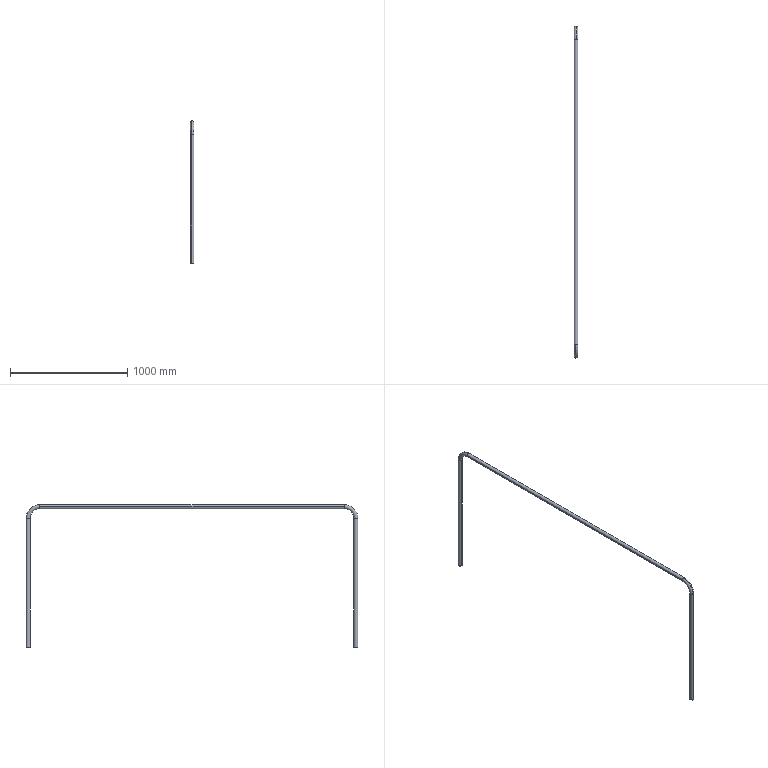Component | SolidWorks | PlatformGuardrail4-1 | 1 solid | 22 faces | box 33.5 x 2833.5 x 1216.75 mm | volume 1470094 mm3 | cylinder 12 | torus 8 | plane 2 | commonest cylinder face diameters 27.5 x6 33.5 x6 | material Plain Carbon Steel
build123d program:
from build123d import *

# Parameters (mm, degrees)
SWEEP_THIN1_PROFILE_R   = 16.75
SWEEP_THIN1_PROFILE_R_2 = 13.75


with BuildPart() as part:
    # Sweep-Thin1: sweep along a path in Sketch1
    with BuildLine(Plane(origin=(0, 0, 0), x_dir=(0, 0, -1), z_dir=(1, 0, 0))) as sweep_thin1_path:
        Line((0, 0), (0, 1100))
        ThreePointArc((0, 1100), (29.289, 1170.711), (100, 1200))
        Line((100, 1200), (2700, 1200))
        ThreePointArc((2700, 1200), (2770.711, 1170.711), (2800, 1100))
        Line((2800, 1100), (2800, 0))
    # Sweep-Thin1 profile (on start of the path) → Sweep-Thin1 (sweep)
    with BuildSketch(Plane.ZX):
        Circle(SWEEP_THIN1_PROFILE_R)
        Circle(SWEEP_THIN1_PROFILE_R_2, mode=Mode.SUBTRACT)
    sweep(path=sweep_thin1_path.line)


solid = part.part

# Placed as in the assembly
solid = solid.moved(Location((6271.051, -551.927, 5590.973), (90, 0, 0)))
STEP:
#1=COLOUR_RGB('',0.7922,0.8196,0.9333);
#2=FILL_AREA_STYLE_COLOUR('',#1);
#3=FILL_AREA_STYLE('',(#2));
#4=SURFACE_STYLE_FILL_AREA(#3);
#5=SURFACE_SIDE_STYLE('',(#4));
#6=SURFACE_STYLE_USAGE(.BOTH.,#5);
#7=PRESENTATION_STYLE_ASSIGNMENT((#6));
#8=CARTESIAN_POINT('',(247.433,84.57,267.361));
#9=VERTEX_POINT('',#8);
#10=CARTESIAN_POINT('',(246.892,84.57,267.902));
#11=VERTEX_POINT('',#10);
#12=CARTESIAN_POINT('',(246.892,84.57,267.361));
#13=DIRECTION('',(-0.,-1.,-0.));
#14=DIRECTION('',(-1.,0.,0.));
#15=AXIS2_PLACEMENT_3D('',#12,#13,#14);
#16=CIRCLE('',#15,0.5413);
#17=EDGE_CURVE('',#9,#11,#16,.T.);
#18=ORIENTED_EDGE('',*,*,#17,.T.);
#19=CARTESIAN_POINT('',(246.892,89.048,263.424));
#20=VERTEX_POINT('',#19);
#21=CARTESIAN_POINT('',(246.892,84.57,263.424));
#22=DIRECTION('',(-1.,0.,-0.));
#23=DIRECTION('',(-0.,-1.,0.));
#24=AXIS2_PLACEMENT_3D('',#21,#22,#23);
#25=CIRCLE('',#24,4.478);
#26=EDGE_CURVE('',#11,#20,#25,.T.);
#27=ORIENTED_EDGE('',*,*,#26,.T.);
#28=CARTESIAN_POINT('',(246.892,87.965,263.424));
#29=VERTEX_POINT('',#28);
#30=CARTESIAN_POINT('',(246.892,88.507,263.424));
#31=DIRECTION('',(-0.,-0.,1.));
#32=DIRECTION('',(-0.,-1.,0.));
#33=AXIS2_PLACEMENT_3D('',#30,#31,#32);
#34=CIRCLE('',#33,0.5413);
#35=EDGE_CURVE('',#29,#20,#34,.T.);
#36=ORIENTED_EDGE('',*,*,#35,.F.);
#37=CARTESIAN_POINT('',(246.892,84.57,266.82));
#38=VERTEX_POINT('',#37);
#39=CARTESIAN_POINT('',(246.892,84.57,263.424));
#40=DIRECTION('',(-1.,0.,-0.));
#41=DIRECTION('',(-0.,-1.,0.));
#42=AXIS2_PLACEMENT_3D('',#39,#40,#41);
#43=CIRCLE('',#42,3.396);
#44=EDGE_CURVE('',#38,#29,#43,.T.);
#45=ORIENTED_EDGE('',*,*,#44,.F.);
#46=CARTESIAN_POINT('',(246.892,84.57,267.361));
#47=DIRECTION('',(-0.,-1.,-0.));
#48=DIRECTION('',(-1.,0.,0.));
#49=AXIS2_PLACEMENT_3D('',#46,#47,#48);
#50=CIRCLE('',#49,0.5413);
#51=EDGE_CURVE('',#38,#9,#50,.T.);
#52=ORIENTED_EDGE('',*,*,#51,.T.);
#53=EDGE_LOOP('',(#18,#27,#36,#45,#52));
#54=FACE_OUTER_BOUND('',#53,.T.);
#55=CARTESIAN_POINT('',(246.892,84.57,263.424));
#56=DIRECTION('',(-1.,0.,-0.));
#57=DIRECTION('',(-0.,-1.,-0.));
#58=AXIS2_PLACEMENT_3D('',#55,#56,#57);
#59=TOROIDAL_SURFACE('',#58,3.937,0.5413);
#60=ADVANCED_FACE('',(#54),#59,.F.);
#61=CARTESIAN_POINT('',(246.892,-21.188,263.424));
#62=VERTEX_POINT('',#61);
#63=CARTESIAN_POINT('',(246.892,-22.271,263.424));
#64=VERTEX_POINT('',#63);
#65=CARTESIAN_POINT('',(246.892,-21.729,263.424));
#66=DIRECTION('',(0.,0.,-1.));
#67=DIRECTION('',(-0.,-1.,0.));
#68=AXIS2_PLACEMENT_3D('',#65,#66,#67);
#69=CIRCLE('',#68,0.5413);
#70=EDGE_CURVE('',#62,#64,#69,.T.);
#71=ORIENTED_EDGE('',*,*,#70,.T.);
#72=CARTESIAN_POINT('',(246.892,-17.792,267.902));
#73=VERTEX_POINT('',#72);
#74=CARTESIAN_POINT('',(246.892,-17.792,263.424));
#75=DIRECTION('',(-1.,0.,-0.));
#76=DIRECTION('',(-0.,-1.,0.));
#77=AXIS2_PLACEMENT_3D('',#74,#75,#76);
#78=CIRCLE('',#77,4.478);
#79=EDGE_CURVE('',#64,#73,#78,.T.);
#80=ORIENTED_EDGE('',*,*,#79,.T.);
#81=CARTESIAN_POINT('',(247.433,-17.792,267.361));
#82=VERTEX_POINT('',#81);
#83=CARTESIAN_POINT('',(246.892,-17.792,267.361));
#84=DIRECTION('',(-0.,-1.,0.));
#85=DIRECTION('',(0.,-0.,-1.));
#86=AXIS2_PLACEMENT_3D('',#83,#84,#85);
#87=CIRCLE('',#86,0.5413);
#88=EDGE_CURVE('',#82,#73,#87,.T.);
#89=ORIENTED_EDGE('',*,*,#88,.F.);
#90=CARTESIAN_POINT('',(246.892,-17.792,266.82));
#91=VERTEX_POINT('',#90);
#92=CARTESIAN_POINT('',(246.892,-17.792,267.361));
#93=DIRECTION('',(-0.,-1.,0.));
#94=DIRECTION('',(0.,-0.,-1.));
#95=AXIS2_PLACEMENT_3D('',#92,#93,#94);
#96=CIRCLE('',#95,0.5413);
#97=EDGE_CURVE('',#91,#82,#96,.T.);
#98=ORIENTED_EDGE('',*,*,#97,.F.);
#99=CARTESIAN_POINT('',(246.892,-17.792,263.424));
#100=DIRECTION('',(-1.,0.,-0.));
#101=DIRECTION('',(-0.,-1.,0.));
#102=AXIS2_PLACEMENT_3D('',#99,#100,#101);
#103=CIRCLE('',#102,3.396);
#104=EDGE_CURVE('',#62,#91,#103,.T.);
#105=ORIENTED_EDGE('',*,*,#104,.F.);
#106=EDGE_LOOP('',(#71,#80,#89,#98,#105));
#107=FACE_OUTER_BOUND('',#106,.T.);
#108=CARTESIAN_POINT('',(246.892,-17.792,263.424));
#109=DIRECTION('',(-1.,0.,-0.));
#110=DIRECTION('',(-0.,-1.,-0.));
#111=AXIS2_PLACEMENT_3D('',#108,#109,#110);
#112=TOROIDAL_SURFACE('',#111,3.937,0.5413);
#113=ADVANCED_FACE('',(#107),#112,.F.);
#114=CARTESIAN_POINT('',(246.892,84.57,268.021));
#115=VERTEX_POINT('',#114);
#116=CARTESIAN_POINT('',(246.232,84.57,267.361));
#117=VERTEX_POINT('',#116);
#118=CARTESIAN_POINT('',(246.892,84.57,267.361));
#119=DIRECTION('',(-0.,-1.,-0.));
#120=DIRECTION('',(0.,0.,-1.));
#121=AXIS2_PLACEMENT_3D('',#118,#119,#120);
#122=CIRCLE('',#121,0.6594);
#123=EDGE_CURVE('',#115,#117,#122,.T.);
#124=ORIENTED_EDGE('',*,*,#123,.F.);
#125=CARTESIAN_POINT('',(246.892,89.166,263.424));
#126=VERTEX_POINT('',#125);
#127=CARTESIAN_POINT('',(246.892,84.57,263.424));
#128=DIRECTION('',(-1.,0.,-0.));
#129=DIRECTION('',(-0.,-1.,0.));
#130=AXIS2_PLACEMENT_3D('',#127,#128,#129);
#131=CIRCLE('',#130,4.596);
#132=EDGE_CURVE('',#115,#126,#131,.T.);
#133=ORIENTED_EDGE('',*,*,#132,.T.);
#134=CARTESIAN_POINT('',(246.892,87.847,263.424));
#135=VERTEX_POINT('',#134);
#136=CARTESIAN_POINT('',(246.892,88.507,263.424));
#137=DIRECTION('',(-0.,-0.,1.));
#138=DIRECTION('',(-0.,-1.,0.));
#139=AXIS2_PLACEMENT_3D('',#136,#137,#138);
#140=CIRCLE('',#139,0.6594);
#141=EDGE_CURVE('',#126,#135,#140,.T.);
#142=ORIENTED_EDGE('',*,*,#141,.T.);
#143=CARTESIAN_POINT('',(246.892,84.57,266.702));
#144=VERTEX_POINT('',#143);
#145=CARTESIAN_POINT('',(246.892,84.57,263.424));
#146=DIRECTION('',(-1.,0.,-0.));
#147=DIRECTION('',(-0.,-1.,0.));
#148=AXIS2_PLACEMENT_3D('',#145,#146,#147);
#149=CIRCLE('',#148,3.278);
#150=EDGE_CURVE('',#144,#135,#149,.T.);
#151=ORIENTED_EDGE('',*,*,#150,.F.);
#152=CARTESIAN_POINT('',(246.892,84.57,267.361));
#153=DIRECTION('',(-0.,-1.,-0.));
#154=DIRECTION('',(0.,0.,-1.));
#155=AXIS2_PLACEMENT_3D('',#152,#153,#154);
#156=CIRCLE('',#155,0.6594);
#157=EDGE_CURVE('',#117,#144,#156,.T.);
#158=ORIENTED_EDGE('',*,*,#157,.F.);
#159=EDGE_LOOP('',(#124,#133,#142,#151,#158));
#160=FACE_OUTER_BOUND('',#159,.T.);
#161=CARTESIAN_POINT('',(246.892,84.57,263.424));
#162=DIRECTION('',(-1.,0.,-0.));
#163=DIRECTION('',(-0.,-1.,0.));
#164=AXIS2_PLACEMENT_3D('',#161,#162,#163);
#165=TOROIDAL_SURFACE('',#164,3.937,0.6594);
#166=ADVANCED_FACE('',(#160),#165,.T.);
#167=CARTESIAN_POINT('',(246.892,-22.389,263.424));
#168=VERTEX_POINT('',#167);
#169=CARTESIAN_POINT('',(246.892,-21.07,263.424));
#170=VERTEX_POINT('',#169);
#171=CARTESIAN_POINT('',(246.892,-21.729,263.424));
#172=DIRECTION('',(0.,0.,-1.));
#173=DIRECTION('',(0.,1.,0.));
#174=AXIS2_PLACEMENT_3D('',#171,#172,#173);
#175=CIRCLE('',#174,0.6594);
#176=EDGE_CURVE('',#168,#170,#175,.T.);
#177=ORIENTED_EDGE('',*,*,#176,.F.);
#178=CARTESIAN_POINT('',(246.892,-17.792,268.021));
#179=VERTEX_POINT('',#178);
#180=CARTESIAN_POINT('',(246.892,-17.792,263.424));
#181=DIRECTION('',(-1.,0.,-0.));
#182=DIRECTION('',(-0.,-1.,0.));
#183=AXIS2_PLACEMENT_3D('',#180,#181,#182);
#184=CIRCLE('',#183,4.596);
#185=EDGE_CURVE('',#168,#179,#184,.T.);
#186=ORIENTED_EDGE('',*,*,#185,.T.);
#187=CARTESIAN_POINT('',(246.232,-17.792,267.361));
#188=VERTEX_POINT('',#187);
#189=CARTESIAN_POINT('',(246.892,-17.792,267.361));
#190=DIRECTION('',(-0.,-1.,0.));
#191=DIRECTION('',(0.,-0.,-1.));
#192=AXIS2_PLACEMENT_3D('',#189,#190,#191);
#193=CIRCLE('',#192,0.6594);
#194=EDGE_CURVE('',#179,#188,#193,.T.);
#195=ORIENTED_EDGE('',*,*,#194,.T.);
#196=CARTESIAN_POINT('',(246.892,-17.792,266.702));
#197=VERTEX_POINT('',#196);
#198=CARTESIAN_POINT('',(246.892,-17.792,267.361));
#199=DIRECTION('',(-0.,-1.,0.));
#200=DIRECTION('',(0.,-0.,-1.));
#201=AXIS2_PLACEMENT_3D('',#198,#199,#200);
#202=CIRCLE('',#201,0.6594);
#203=EDGE_CURVE('',#188,#197,#202,.T.);
#204=ORIENTED_EDGE('',*,*,#203,.T.);
#205=CARTESIAN_POINT('',(246.892,-17.792,263.424));
#206=DIRECTION('',(-1.,0.,-0.));
#207=DIRECTION('',(-0.,-1.,0.));
#208=AXIS2_PLACEMENT_3D('',#205,#206,#207);
#209=CIRCLE('',#208,3.278);
#210=EDGE_CURVE('',#170,#197,#209,.T.);
#211=ORIENTED_EDGE('',*,*,#210,.F.);
#212=EDGE_LOOP('',(#177,#186,#195,#204,#211));
#213=FACE_OUTER_BOUND('',#212,.T.);
#214=CARTESIAN_POINT('',(246.892,-17.792,263.424));
#215=DIRECTION('',(-1.,0.,-0.));
#216=DIRECTION('',(-0.,-1.,0.));
#217=AXIS2_PLACEMENT_3D('',#214,#215,#216);
#218=TOROIDAL_SURFACE('',#217,3.937,0.6594);
#219=ADVANCED_FACE('',(#213),#218,.T.);
#220=CARTESIAN_POINT('',(246.892,88.507,263.424));
#221=DIRECTION('',(-0.,-0.,1.));
#222=DIRECTION('',(-0.,-1.,0.));
#223=AXIS2_PLACEMENT_3D('',#220,#221,#222);
#224=CIRCLE('',#223,0.5413);
#225=EDGE_CURVE('',#20,#29,#224,.T.);
#226=ORIENTED_EDGE('',*,*,#225,.T.);
#227=CARTESIAN_POINT('',(246.892,87.965,220.117));
#228=VERTEX_POINT('',#227);
#229=CARTESIAN_POINT('',(246.892,87.965,263.424));
#230=DIRECTION('',(0.,0.,-1.));
#231=VECTOR('',#230,39.37);
#232=LINE('',#229,#231);
#233=EDGE_CURVE('',#29,#228,#232,.T.);
#234=ORIENTED_EDGE('',*,*,#233,.T.);
#235=CARTESIAN_POINT('',(246.892,89.048,220.117));
#236=VERTEX_POINT('',#235);
#237=CARTESIAN_POINT('',(246.892,88.507,220.117));
#238=DIRECTION('',(-0.,-0.,1.));
#239=DIRECTION('',(-0.,-1.,0.));
#240=AXIS2_PLACEMENT_3D('',#237,#238,#239);
#241=CIRCLE('',#240,0.5413);
#242=EDGE_CURVE('',#236,#228,#241,.T.);
#243=ORIENTED_EDGE('',*,*,#242,.F.);
#244=CARTESIAN_POINT('',(246.892,89.048,263.424));
#245=DIRECTION('',(0.,0.,-1.));
#246=VECTOR('',#245,39.37);
#247=LINE('',#244,#246);
#248=EDGE_CURVE('',#20,#236,#247,.T.);
#249=ORIENTED_EDGE('',*,*,#248,.F.);
#250=EDGE_LOOP('',(#226,#234,#243,#249));
#251=FACE_OUTER_BOUND('',#250,.T.);
#252=CARTESIAN_POINT('',(246.892,88.507,263.424));
#253=DIRECTION('',(0.,0.,-1.));
#254=DIRECTION('',(0.,1.,0.));
#255=AXIS2_PLACEMENT_3D('',#252,#253,#254);
#256=CYLINDRICAL_SURFACE('',#255,0.5413);
#257=ADVANCED_FACE('',(#251),#256,.F.);
#258=CARTESIAN_POINT('',(246.35,-17.792,267.361));
#259=VERTEX_POINT('',#258);
#260=CARTESIAN_POINT('',(246.892,-17.792,267.361));
#261=DIRECTION('',(-0.,-1.,0.));
#262=DIRECTION('',(0.,-0.,-1.));
#263=AXIS2_PLACEMENT_3D('',#260,#261,#262);
#264=CIRCLE('',#263,0.5413);
#265=EDGE_CURVE('',#259,#91,#264,.T.);
#266=ORIENTED_EDGE('',*,*,#265,.T.);
#267=ORIENTED_EDGE('',*,*,#97,.T.);
#268=CARTESIAN_POINT('',(247.433,-17.792,267.361));
#269=DIRECTION('',(0.,1.,0.));
#270=VECTOR('',#269,39.37);
#271=LINE('',#268,#270);
#272=EDGE_CURVE('',#82,#9,#271,.T.);
#273=ORIENTED_EDGE('',*,*,#272,.T.);
#274=ORIENTED_EDGE('',*,*,#51,.F.);
#275=CARTESIAN_POINT('',(246.35,84.57,267.361));
#276=VERTEX_POINT('',#275);
#277=CARTESIAN_POINT('',(246.892,84.57,267.361));
#278=DIRECTION('',(-0.,-1.,-0.));
#279=DIRECTION('',(-1.,0.,0.));
#280=AXIS2_PLACEMENT_3D('',#277,#278,#279);
#281=CIRCLE('',#280,0.5413);
#282=EDGE_CURVE('',#276,#38,#281,.T.);
#283=ORIENTED_EDGE('',*,*,#282,.F.);
#284=CARTESIAN_POINT('',(246.35,-17.792,267.361));
#285=DIRECTION('',(0.,1.,0.));
#286=VECTOR('',#285,39.37);
#287=LINE('',#284,#286);
#288=EDGE_CURVE('',#259,#276,#287,.T.);
#289=ORIENTED_EDGE('',*,*,#288,.F.);
#290=EDGE_LOOP('',(#266,#267,#273,#274,#283,#289));
#291=FACE_OUTER_BOUND('',#290,.T.);
#292=CARTESIAN_POINT('',(246.892,-17.792,267.361));
#293=DIRECTION('',(0.,1.,0.));
#294=DIRECTION('',(-1.,0.,0.));
#295=AXIS2_PLACEMENT_3D('',#292,#293,#294);
#296=CYLINDRICAL_SURFACE('',#295,0.5413);
#297=ADVANCED_FACE('',(#291),#296,.F.);
#298=CARTESIAN_POINT('',(246.892,-22.271,220.117));
#299=VERTEX_POINT('',#298);
#300=CARTESIAN_POINT('',(246.892,-21.188,220.117));
#301=VERTEX_POINT('',#300);
#302=CARTESIAN_POINT('',(246.892,-21.729,220.117));
#303=DIRECTION('',(0.,0.,-1.));
#304=DIRECTION('',(0.,1.,0.));
#305=AXIS2_PLACEMENT_3D('',#302,#303,#304);
#306=CIRCLE('',#305,0.5413);
#307=EDGE_CURVE('',#299,#301,#306,.T.);
#308=ORIENTED_EDGE('',*,*,#307,.T.);
#309=CARTESIAN_POINT('',(246.892,-21.188,220.117));
#310=DIRECTION('',(-0.,-0.,1.));
#311=VECTOR('',#310,39.37);
#312=LINE('',#309,#311);
#313=EDGE_CURVE('',#301,#62,#312,.T.);
#314=ORIENTED_EDGE('',*,*,#313,.T.);
#315=CARTESIAN_POINT('',(246.892,-21.729,263.424));
#316=DIRECTION('',(0.,0.,-1.));
#317=DIRECTION('',(-0.,-1.,0.));
#318=AXIS2_PLACEMENT_3D('',#315,#316,#317);
#319=CIRCLE('',#318,0.5413);
#320=EDGE_CURVE('',#64,#62,#319,.T.);
#321=ORIENTED_EDGE('',*,*,#320,.F.);
#322=CARTESIAN_POINT('',(246.892,-22.271,220.117));
#323=DIRECTION('',(-0.,-0.,1.));
#324=VECTOR('',#323,39.37);
#325=LINE('',#322,#324);
#326=EDGE_CURVE('',#299,#64,#325,.T.);
#327=ORIENTED_EDGE('',*,*,#326,.F.);
#328=EDGE_LOOP('',(#308,#314,#321,#327));
#329=FACE_OUTER_BOUND('',#328,.T.);
#330=CARTESIAN_POINT('',(246.892,-21.729,220.117));
#331=DIRECTION('',(-0.,-0.,1.));
#332=DIRECTION('',(-0.,-1.,0.));
#333=AXIS2_PLACEMENT_3D('',#330,#331,#332);
#334=CYLINDRICAL_SURFACE('',#333,0.5413);
#335=ADVANCED_FACE('',(#329),#334,.F.);
#336=CARTESIAN_POINT('',(246.892,88.507,263.424));
#337=DIRECTION('',(-0.,-0.,1.));
#338=DIRECTION('',(-0.,-1.,0.));
#339=AXIS2_PLACEMENT_3D('',#336,#337,#338);
#340=CIRCLE('',#339,0.6594);
#341=EDGE_CURVE('',#135,#126,#340,.T.);
#342=ORIENTED_EDGE('',*,*,#341,.F.);
#343=CARTESIAN_POINT('',(246.892,87.847,220.117));
#344=VERTEX_POINT('',#343);
#345=CARTESIAN_POINT('',(246.892,87.847,263.424));
#346=DIRECTION('',(0.,0.,-1.));
#347=VECTOR('',#346,39.37);
#348=LINE('',#345,#347);
#349=EDGE_CURVE('',#135,#344,#348,.T.);
#350=ORIENTED_EDGE('',*,*,#349,.T.);
#351=CARTESIAN_POINT('',(246.892,89.166,220.117));
#352=VERTEX_POINT('',#351);
#353=CARTESIAN_POINT('',(246.892,88.507,220.117));
#354=DIRECTION('',(-0.,-0.,1.));
#355=DIRECTION('',(-0.,-1.,0.));
#356=AXIS2_PLACEMENT_3D('',#353,#354,#355);
#357=CIRCLE('',#356,0.6594);
#358=EDGE_CURVE('',#344,#352,#357,.T.);
#359=ORIENTED_EDGE('',*,*,#358,.T.);
#360=CARTESIAN_POINT('',(246.892,89.166,263.424));
#361=DIRECTION('',(0.,0.,-1.));
#362=VECTOR('',#361,39.37);
#363=LINE('',#360,#362);
#364=EDGE_CURVE('',#126,#352,#363,.T.);
#365=ORIENTED_EDGE('',*,*,#364,.F.);
#366=EDGE_LOOP('',(#342,#350,#359,#365));
#367=FACE_OUTER_BOUND('',#366,.T.);
#368=CARTESIAN_POINT('',(246.892,88.507,263.424));
#369=DIRECTION('',(0.,0.,-1.));
#370=DIRECTION('',(0.,1.,0.));
#371=AXIS2_PLACEMENT_3D('',#368,#369,#370);
#372=CYLINDRICAL_SURFACE('',#371,0.6594);
#373=ADVANCED_FACE('',(#367),#372,.T.);
#374=CARTESIAN_POINT('',(247.551,-17.792,267.361));
#375=VERTEX_POINT('',#374);
#376=CARTESIAN_POINT('',(246.892,-17.792,267.361));
#377=DIRECTION('',(-0.,-1.,0.));
#378=DIRECTION('',(0.,-0.,-1.));
#379=AXIS2_PLACEMENT_3D('',#376,#377,#378);
#380=CIRCLE('',#379,0.6594);
#381=EDGE_CURVE('',#375,#179,#380,.T.);
#382=ORIENTED_EDGE('',*,*,#381,.F.);
#383=CARTESIAN_POINT('',(247.551,84.57,267.361));
#384=VERTEX_POINT('',#383);
#385=CARTESIAN_POINT('',(247.551,-17.792,267.361));
#386=DIRECTION('',(0.,1.,0.));
#387=VECTOR('',#386,39.37);
#388=LINE('',#385,#387);
#389=EDGE_CURVE('',#375,#384,#388,.T.);
#390=ORIENTED_EDGE('',*,*,#389,.T.);
#391=CARTESIAN_POINT('',(246.892,84.57,267.361));
#392=DIRECTION('',(-0.,-1.,-0.));
#393=DIRECTION('',(0.,0.,-1.));
#394=AXIS2_PLACEMENT_3D('',#391,#392,#393);
#395=CIRCLE('',#394,0.6594);
#396=EDGE_CURVE('',#384,#115,#395,.T.);
#397=ORIENTED_EDGE('',*,*,#396,.T.);
#398=ORIENTED_EDGE('',*,*,#123,.T.);
#399=CARTESIAN_POINT('',(246.232,-17.792,267.361));
#400=DIRECTION('',(0.,1.,0.));
#401=VECTOR('',#400,39.37);
#402=LINE('',#399,#401);
#403=EDGE_CURVE('',#188,#117,#402,.T.);
#404=ORIENTED_EDGE('',*,*,#403,.F.);
#405=ORIENTED_EDGE('',*,*,#194,.F.);
#406=EDGE_LOOP('',(#382,#390,#397,#398,#404,#405));
#407=FACE_OUTER_BOUND('',#406,.T.);
#408=CARTESIAN_POINT('',(246.892,-17.792,267.361));
#409=DIRECTION('',(0.,1.,0.));
#410=DIRECTION('',(-1.,0.,0.));
#411=AXIS2_PLACEMENT_3D('',#408,#409,#410);
#412=CYLINDRICAL_SURFACE('',#411,0.6594);
#413=ADVANCED_FACE('',(#407),#412,.T.);
#414=CARTESIAN_POINT('',(246.892,-21.07,220.117));
#415=VERTEX_POINT('',#414);
#416=CARTESIAN_POINT('',(246.892,-22.389,220.117));
#417=VERTEX_POINT('',#416);
#418=CARTESIAN_POINT('',(246.892,-21.729,220.117));
#419=DIRECTION('',(0.,0.,-1.));
#420=DIRECTION('',(0.,1.,0.));
#421=AXIS2_PLACEMENT_3D('',#418,#419,#420);
#422=CIRCLE('',#421,0.6594);
#423=EDGE_CURVE('',#415,#417,#422,.T.);
#424=ORIENTED_EDGE('',*,*,#423,.F.);
#425=CARTESIAN_POINT('',(246.892,-21.07,220.117));
#426=DIRECTION('',(-0.,-0.,1.));
#427=VECTOR('',#426,39.37);
#428=LINE('',#425,#427);
#429=EDGE_CURVE('',#415,#170,#428,.T.);
#430=ORIENTED_EDGE('',*,*,#429,.T.);
#431=CARTESIAN_POINT('',(246.892,-21.729,263.424));
#432=DIRECTION('',(0.,0.,-1.));
#433=DIRECTION('',(0.,1.,0.));
#434=AXIS2_PLACEMENT_3D('',#431,#432,#433);
#435=CIRCLE('',#434,0.6594);
#436=EDGE_CURVE('',#170,#168,#435,.T.);
#437=ORIENTED_EDGE('',*,*,#436,.T.);
#438=CARTESIAN_POINT('',(246.892,-22.389,220.117));
#439=DIRECTION('',(-0.,-0.,1.));
#440=VECTOR('',#439,39.37);
#441=LINE('',#438,#440);
#442=EDGE_CURVE('',#417,#168,#441,.T.);
#443=ORIENTED_EDGE('',*,*,#442,.F.);
#444=EDGE_LOOP('',(#424,#430,#437,#443));
#445=FACE_OUTER_BOUND('',#444,.T.);
#446=CARTESIAN_POINT('',(246.892,-21.729,220.117));
#447=DIRECTION('',(-0.,-0.,1.));
#448=DIRECTION('',(-0.,-1.,0.));
#449=AXIS2_PLACEMENT_3D('',#446,#447,#448);
#450=CYLINDRICAL_SURFACE('',#449,0.6594);
#451=ADVANCED_FACE('',(#445),#450,.T.);
#452=ORIENTED_EDGE('',*,*,#349,.F.);
#453=ORIENTED_EDGE('',*,*,#141,.F.);
#454=ORIENTED_EDGE('',*,*,#364,.T.);
#455=CARTESIAN_POINT('',(246.892,88.507,220.117));
#456=DIRECTION('',(-0.,-0.,1.));
#457=DIRECTION('',(-0.,-1.,0.));
#458=AXIS2_PLACEMENT_3D('',#455,#456,#457);
#459=CIRCLE('',#458,0.6594);
#460=EDGE_CURVE('',#352,#344,#459,.T.);
#461=ORIENTED_EDGE('',*,*,#460,.T.);
#462=EDGE_LOOP('',(#452,#453,#454,#461));
#463=FACE_OUTER_BOUND('',#462,.T.);
#464=CARTESIAN_POINT('',(246.892,88.507,263.424));
#465=DIRECTION('',(0.,0.,-1.));
#466=DIRECTION('',(0.,1.,0.));
#467=AXIS2_PLACEMENT_3D('',#464,#465,#466);
#468=CYLINDRICAL_SURFACE('',#467,0.6594);
#469=ADVANCED_FACE('',(#463),#468,.T.);
#470=ORIENTED_EDGE('',*,*,#132,.F.);
#471=ORIENTED_EDGE('',*,*,#396,.F.);
#472=CARTESIAN_POINT('',(246.892,84.57,267.361));
#473=DIRECTION('',(-0.,-1.,-0.));
#474=DIRECTION('',(0.,0.,-1.));
#475=AXIS2_PLACEMENT_3D('',#472,#473,#474);
#476=CIRCLE('',#475,0.6594);
#477=EDGE_CURVE('',#144,#384,#476,.T.);
#478=ORIENTED_EDGE('',*,*,#477,.F.);
#479=ORIENTED_EDGE('',*,*,#150,.T.);
#480=ORIENTED_EDGE('',*,*,#341,.T.);
#481=EDGE_LOOP('',(#470,#471,#478,#479,#480));
#482=FACE_OUTER_BOUND('',#481,.T.);
#483=CARTESIAN_POINT('',(246.892,84.57,263.424));
#484=DIRECTION('',(-1.,0.,-0.));
#485=DIRECTION('',(-0.,-1.,0.));
#486=AXIS2_PLACEMENT_3D('',#483,#484,#485);
#487=TOROIDAL_SURFACE('',#486,3.937,0.6594);
#488=ADVANCED_FACE('',(#482),#487,.T.);
#489=ORIENTED_EDGE('',*,*,#389,.F.);
#490=CARTESIAN_POINT('',(246.892,-17.792,267.361));
#491=DIRECTION('',(-0.,-1.,0.));
#492=DIRECTION('',(0.,-0.,-1.));
#493=AXIS2_PLACEMENT_3D('',#490,#491,#492);
#494=CIRCLE('',#493,0.6594);
#495=EDGE_CURVE('',#197,#375,#494,.T.);
#496=ORIENTED_EDGE('',*,*,#495,.F.);
#497=ORIENTED_EDGE('',*,*,#203,.F.);
#498=ORIENTED_EDGE('',*,*,#403,.T.);
#499=ORIENTED_EDGE('',*,*,#157,.T.);
#500=ORIENTED_EDGE('',*,*,#477,.T.);
#501=EDGE_LOOP('',(#489,#496,#497,#498,#499,#500));
#502=FACE_OUTER_BOUND('',#501,.T.);
#503=CARTESIAN_POINT('',(246.892,-17.792,267.361));
#504=DIRECTION('',(0.,1.,0.));
#505=DIRECTION('',(-1.,0.,0.));
#506=AXIS2_PLACEMENT_3D('',#503,#504,#505);
#507=CYLINDRICAL_SURFACE('',#506,0.6594);
#508=ADVANCED_FACE('',(#502),#507,.T.);
#509=ORIENTED_EDGE('',*,*,#185,.F.);
#510=ORIENTED_EDGE('',*,*,#436,.F.);
#511=ORIENTED_EDGE('',*,*,#210,.T.);
#512=ORIENTED_EDGE('',*,*,#495,.T.);
#513=ORIENTED_EDGE('',*,*,#381,.T.);
#514=EDGE_LOOP('',(#509,#510,#511,#512,#513));
#515=FACE_OUTER_BOUND('',#514,.T.);
#516=CARTESIAN_POINT('',(246.892,-17.792,263.424));
#517=DIRECTION('',(-1.,0.,-0.));
#518=DIRECTION('',(-0.,-1.,0.));
#519=AXIS2_PLACEMENT_3D('',#516,#517,#518);
#520=TOROIDAL_SURFACE('',#519,3.937,0.6594);
#521=ADVANCED_FACE('',(#515),#520,.T.);
#522=ORIENTED_EDGE('',*,*,#429,.F.);
#523=CARTESIAN_POINT('',(246.892,-21.729,220.117));
#524=DIRECTION('',(0.,0.,-1.));
#525=DIRECTION('',(0.,1.,0.));
#526=AXIS2_PLACEMENT_3D('',#523,#524,#525);
#527=CIRCLE('',#526,0.6594);
#528=EDGE_CURVE('',#417,#415,#527,.T.);
#529=ORIENTED_EDGE('',*,*,#528,.F.);
#530=ORIENTED_EDGE('',*,*,#442,.T.);
#531=ORIENTED_EDGE('',*,*,#176,.T.);
#532=EDGE_LOOP('',(#522,#529,#530,#531));
#533=FACE_OUTER_BOUND('',#532,.T.);
#534=CARTESIAN_POINT('',(246.892,-21.729,220.117));
#535=DIRECTION('',(-0.,-0.,1.));
#536=DIRECTION('',(-0.,-1.,0.));
#537=AXIS2_PLACEMENT_3D('',#534,#535,#536);
#538=CYLINDRICAL_SURFACE('',#537,0.6594);
#539=ADVANCED_FACE('',(#533),#538,.T.);
#540=ORIENTED_EDGE('',*,*,#242,.T.);
#541=CARTESIAN_POINT('',(246.892,88.507,220.117));
#542=DIRECTION('',(-0.,-0.,1.));
#543=DIRECTION('',(-0.,-1.,0.));
#544=AXIS2_PLACEMENT_3D('',#541,#542,#543);
#545=CIRCLE('',#544,0.5413);
#546=EDGE_CURVE('',#228,#236,#545,.T.);
#547=ORIENTED_EDGE('',*,*,#546,.T.);
#548=EDGE_LOOP('',(#540,#547));
#549=FACE_BOUND('',#548,.T.);
#550=ORIENTED_EDGE('',*,*,#460,.F.);
#551=ORIENTED_EDGE('',*,*,#358,.F.);
#552=EDGE_LOOP('',(#550,#551));
#553=FACE_OUTER_BOUND('',#552,.T.);
#554=CARTESIAN_POINT('',(246.892,88.507,220.117));
#555=DIRECTION('',(-0.,-0.,1.));
#556=DIRECTION('',(-0.,-1.,-0.));
#557=AXIS2_PLACEMENT_3D('',#554,#555,#556);
#558=PLANE('',#557);
#559=ADVANCED_FACE('',(#549,#553),#558,.F.);
#560=ORIENTED_EDGE('',*,*,#307,.F.);
#561=CARTESIAN_POINT('',(246.892,-21.729,220.117));
#562=DIRECTION('',(0.,0.,-1.));
#563=DIRECTION('',(0.,1.,0.));
#564=AXIS2_PLACEMENT_3D('',#561,#562,#563);
#565=CIRCLE('',#564,0.5413);
#566=EDGE_CURVE('',#301,#299,#565,.T.);
#567=ORIENTED_EDGE('',*,*,#566,.F.);
#568=EDGE_LOOP('',(#560,#567));
#569=FACE_BOUND('',#568,.T.);
#570=ORIENTED_EDGE('',*,*,#528,.T.);
#571=ORIENTED_EDGE('',*,*,#423,.T.);
#572=EDGE_LOOP('',(#570,#571));
#573=FACE_OUTER_BOUND('',#572,.T.);
#574=CARTESIAN_POINT('',(246.892,-21.729,220.117));
#575=DIRECTION('',(0.,0.,-1.));
#576=DIRECTION('',(0.,1.,0.));
#577=AXIS2_PLACEMENT_3D('',#574,#575,#576);
#578=PLANE('',#577);
#579=ADVANCED_FACE('',(#569,#573),#578,.T.);
#580=ORIENTED_EDGE('',*,*,#233,.F.);
#581=ORIENTED_EDGE('',*,*,#35,.T.);
#582=ORIENTED_EDGE('',*,*,#248,.T.);
#583=ORIENTED_EDGE('',*,*,#546,.F.);
#584=EDGE_LOOP('',(#580,#581,#582,#583));
#585=FACE_OUTER_BOUND('',#584,.T.);
#586=CARTESIAN_POINT('',(246.892,88.507,263.424));
#587=DIRECTION('',(0.,0.,-1.));
#588=DIRECTION('',(0.,1.,0.));
#589=AXIS2_PLACEMENT_3D('',#586,#587,#588);
#590=CYLINDRICAL_SURFACE('',#589,0.5413);
#591=ADVANCED_FACE('',(#585),#590,.F.);
#592=ORIENTED_EDGE('',*,*,#26,.F.);
#593=CARTESIAN_POINT('',(246.892,84.57,267.361));
#594=DIRECTION('',(-0.,-1.,-0.));
#595=DIRECTION('',(-1.,0.,0.));
#596=AXIS2_PLACEMENT_3D('',#593,#594,#595);
#597=CIRCLE('',#596,0.5413);
#598=EDGE_CURVE('',#11,#276,#597,.T.);
#599=ORIENTED_EDGE('',*,*,#598,.T.);
#600=ORIENTED_EDGE('',*,*,#282,.T.);
#601=ORIENTED_EDGE('',*,*,#44,.T.);
#602=ORIENTED_EDGE('',*,*,#225,.F.);
#603=EDGE_LOOP('',(#592,#599,#600,#601,#602));
#604=FACE_OUTER_BOUND('',#603,.T.);
#605=CARTESIAN_POINT('',(246.892,84.57,263.424));
#606=DIRECTION('',(-1.,0.,-0.));
#607=DIRECTION('',(-0.,-1.,-0.));
#608=AXIS2_PLACEMENT_3D('',#605,#606,#607);
#609=TOROIDAL_SURFACE('',#608,3.937,0.5413);
#610=ADVANCED_FACE('',(#604),#609,.F.);
#611=ORIENTED_EDGE('',*,*,#272,.F.);
#612=ORIENTED_EDGE('',*,*,#88,.T.);
#613=CARTESIAN_POINT('',(246.892,-17.792,267.361));
#614=DIRECTION('',(-0.,-1.,0.));
#615=DIRECTION('',(0.,-0.,-1.));
#616=AXIS2_PLACEMENT_3D('',#613,#614,#615);
#617=CIRCLE('',#616,0.5413);
#618=EDGE_CURVE('',#73,#259,#617,.T.);
#619=ORIENTED_EDGE('',*,*,#618,.T.);
#620=ORIENTED_EDGE('',*,*,#288,.T.);
#621=ORIENTED_EDGE('',*,*,#598,.F.);
#622=ORIENTED_EDGE('',*,*,#17,.F.);
#623=EDGE_LOOP('',(#611,#612,#619,#620,#621,#622));
#624=FACE_OUTER_BOUND('',#623,.T.);
#625=CARTESIAN_POINT('',(246.892,-17.792,267.361));
#626=DIRECTION('',(0.,1.,0.));
#627=DIRECTION('',(-1.,0.,0.));
#628=AXIS2_PLACEMENT_3D('',#625,#626,#627);
#629=CYLINDRICAL_SURFACE('',#628,0.5413);
#630=ADVANCED_FACE('',(#624),#629,.F.);
#631=ORIENTED_EDGE('',*,*,#79,.F.);
#632=ORIENTED_EDGE('',*,*,#320,.T.);
#633=ORIENTED_EDGE('',*,*,#104,.T.);
#634=ORIENTED_EDGE('',*,*,#265,.F.);
#635=ORIENTED_EDGE('',*,*,#618,.F.);
#636=EDGE_LOOP('',(#631,#632,#633,#634,#635));
#637=FACE_OUTER_BOUND('',#636,.T.);
#638=CARTESIAN_POINT('',(246.892,-17.792,263.424));
#639=DIRECTION('',(-1.,0.,-0.));
#640=DIRECTION('',(-0.,-1.,-0.));
#641=AXIS2_PLACEMENT_3D('',#638,#639,#640);
#642=TOROIDAL_SURFACE('',#641,3.937,0.5413);
#643=ADVANCED_FACE('',(#637),#642,.F.);
#644=ORIENTED_EDGE('',*,*,#313,.F.);
#645=ORIENTED_EDGE('',*,*,#566,.T.);
#646=ORIENTED_EDGE('',*,*,#326,.T.);
#647=ORIENTED_EDGE('',*,*,#70,.F.);
#648=EDGE_LOOP('',(#644,#645,#646,#647));
#649=FACE_OUTER_BOUND('',#648,.T.);
#650=CARTESIAN_POINT('',(246.892,-21.729,220.117));
#651=DIRECTION('',(-0.,-0.,1.));
#652=DIRECTION('',(-0.,-1.,0.));
#653=AXIS2_PLACEMENT_3D('',#650,#651,#652);
#654=CYLINDRICAL_SURFACE('',#653,0.5413);
#655=ADVANCED_FACE('',(#649),#654,.F.);
#656=CLOSED_SHELL('',(#60,#113,#166,#219,#257,#297,#335,#373,#413,#451,#469,#488,#508,#521,#539,#559,#579,#591,#610,#630,#643,#655));
#657=MANIFOLD_SOLID_BREP('',#656);
#658=STYLED_ITEM('',(#7),#657);
#659=(LENGTH_UNIT()NAMED_UNIT(*)SI_UNIT($,.METRE.));
#660=LENGTH_MEASURE_WITH_UNIT(LENGTH_MEASURE(0.0254),#659);
#661=DIMENSIONAL_EXPONENTS(1.,0.,0.,0.,0.,0.,0.);
#662=(CONVERSION_BASED_UNIT('',#660)LENGTH_UNIT()NAMED_UNIT(#661));
#663=UNCERTAINTY_MEASURE_WITH_UNIT(LENGTH_MEASURE(0.00001),#662,'','');
#664=(NAMED_UNIT(*)PLANE_ANGLE_UNIT()SI_UNIT($,.RADIAN.));
#665=(NAMED_UNIT(*)SI_UNIT($,.STERADIAN.)SOLID_ANGLE_UNIT());
#666=(GEOMETRIC_REPRESENTATION_CONTEXT(3)GLOBAL_UNCERTAINTY_ASSIGNED_CONTEXT((#663))GLOBAL_UNIT_ASSIGNED_CONTEXT((#662,#664,#665))REPRESENTATION_CONTEXT('',''));
#667=MECHANICAL_DESIGN_GEOMETRIC_PRESENTATION_REPRESENTATION('',(#658),#666);
#668=PRESENTATION_LAYER_ASSIGNMENT('','',(#658));
#669=CARTESIAN_POINT('',(0.,0.,0.));
#670=DIRECTION('',(0.,0.,1.));
#671=DIRECTION('',(1.,0.,0.));
#672=AXIS2_PLACEMENT_3D('',#669,#670,#671);
#673=(LENGTH_UNIT()NAMED_UNIT(*)SI_UNIT($,.METRE.));
#674=LENGTH_MEASURE_WITH_UNIT(LENGTH_MEASURE(0.0254),#673);
#675=DIMENSIONAL_EXPONENTS(1.,0.,0.,0.,0.,0.,0.);
#676=(CONVERSION_BASED_UNIT('',#674)LENGTH_UNIT()NAMED_UNIT(#675));
#677=UNCERTAINTY_MEASURE_WITH_UNIT(LENGTH_MEASURE(0.00001),#676,'','');
#678=(NAMED_UNIT(*)PLANE_ANGLE_UNIT()SI_UNIT($,.RADIAN.));
#679=(NAMED_UNIT(*)SI_UNIT($,.STERADIAN.)SOLID_ANGLE_UNIT());
#680=(GEOMETRIC_REPRESENTATION_CONTEXT(3)GLOBAL_UNCERTAINTY_ASSIGNED_CONTEXT((#677))GLOBAL_UNIT_ASSIGNED_CONTEXT((#676,#678,#679))REPRESENTATION_CONTEXT('',''));
#681=ADVANCED_BREP_SHAPE_REPRESENTATION('',(#657,#672),#680);